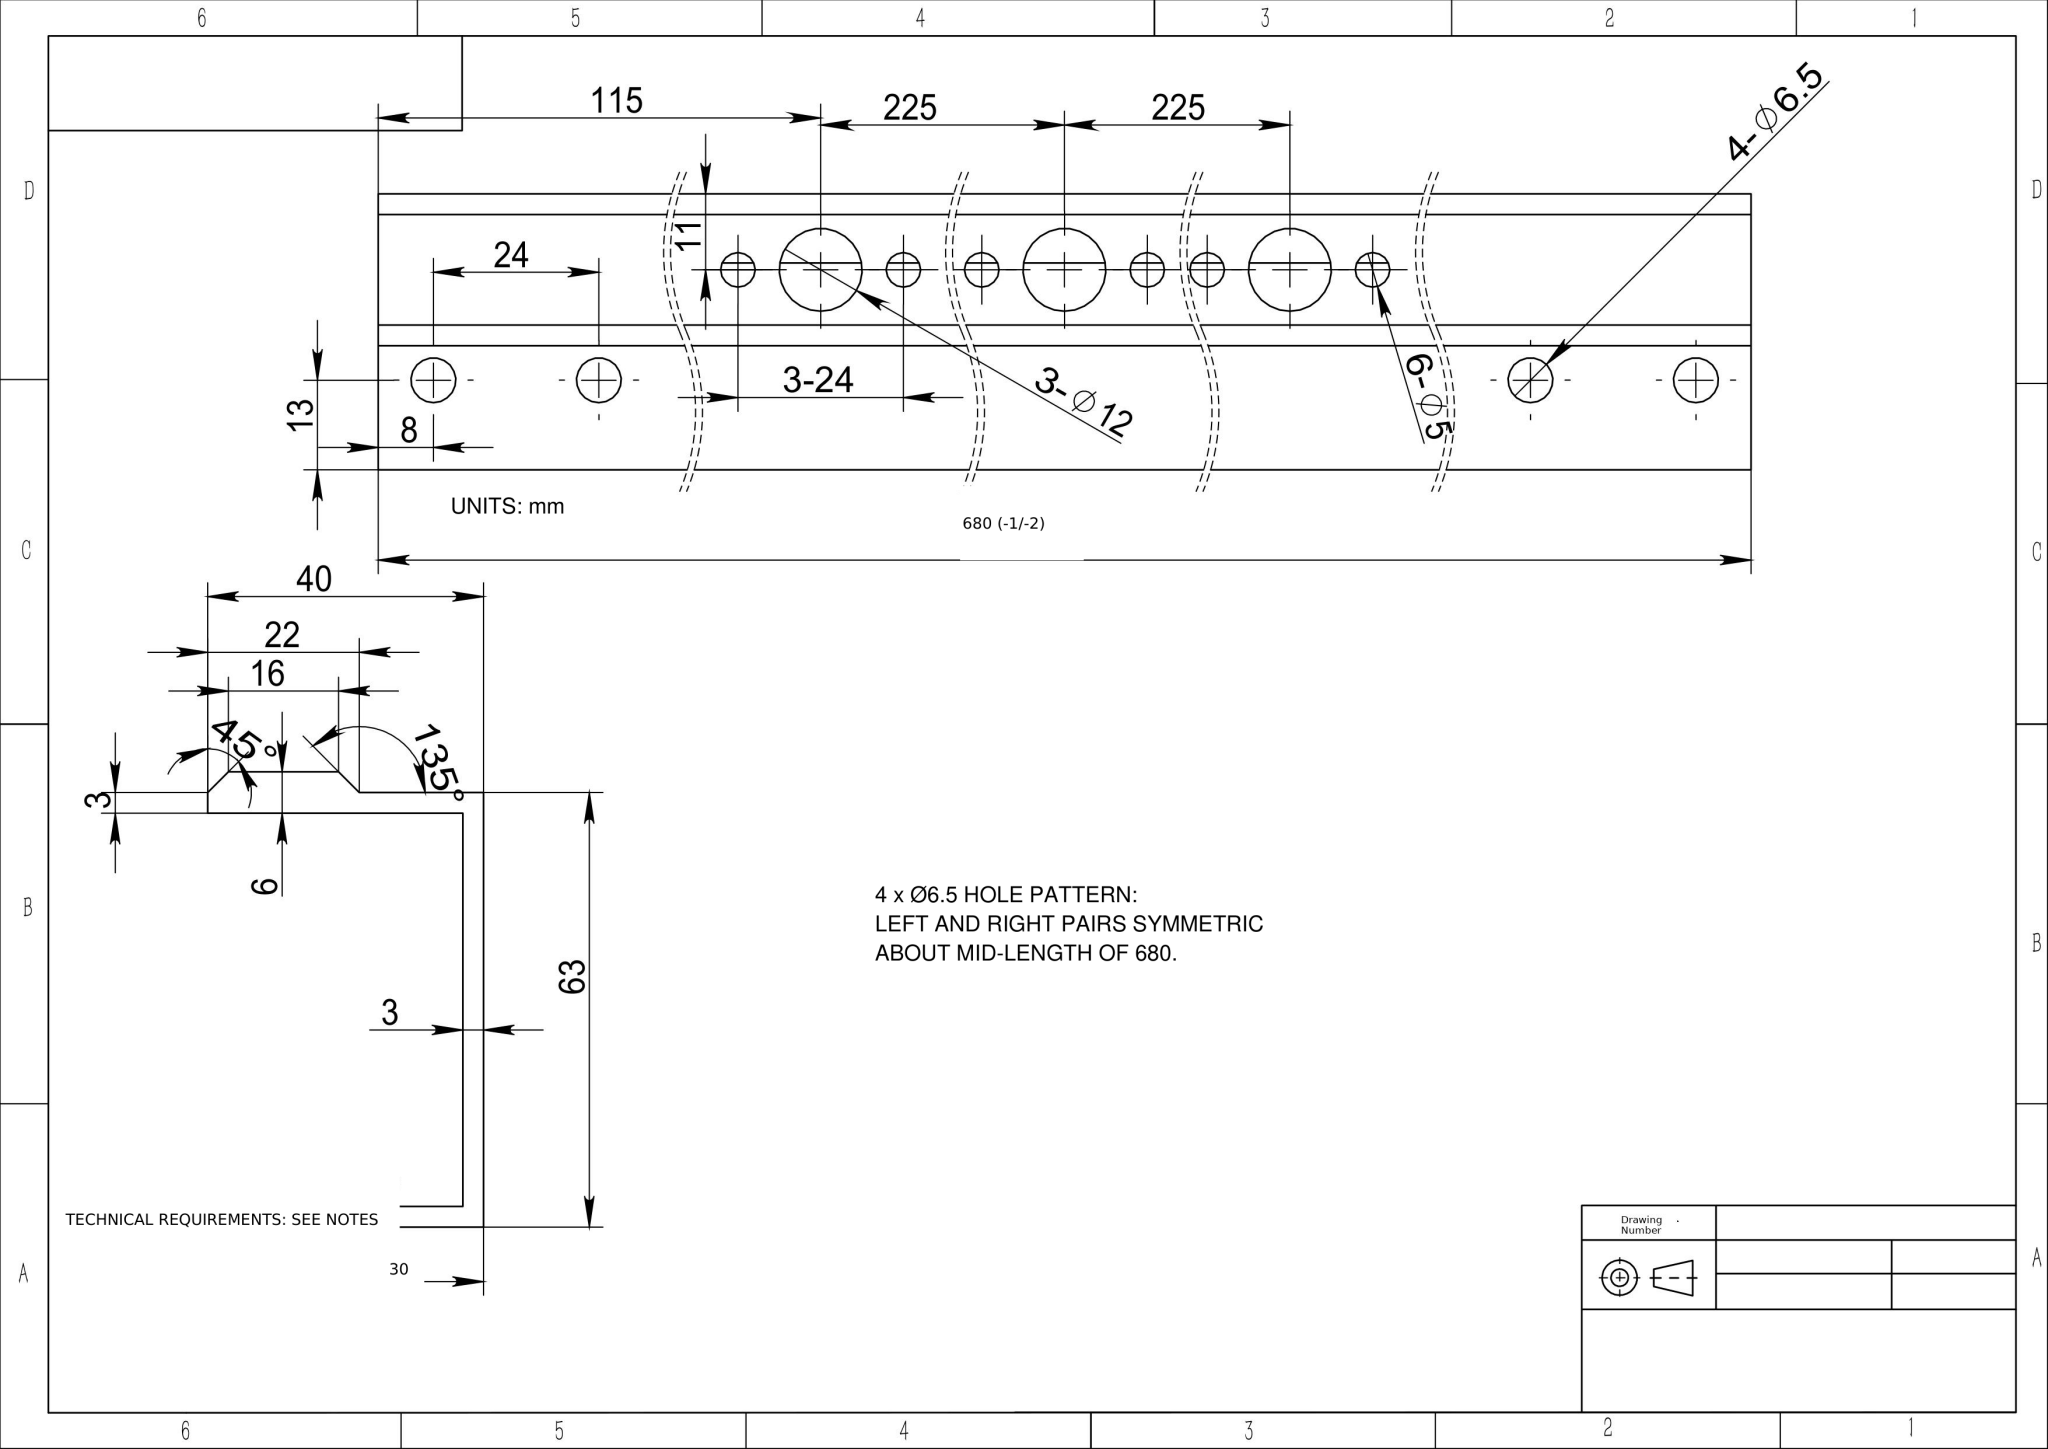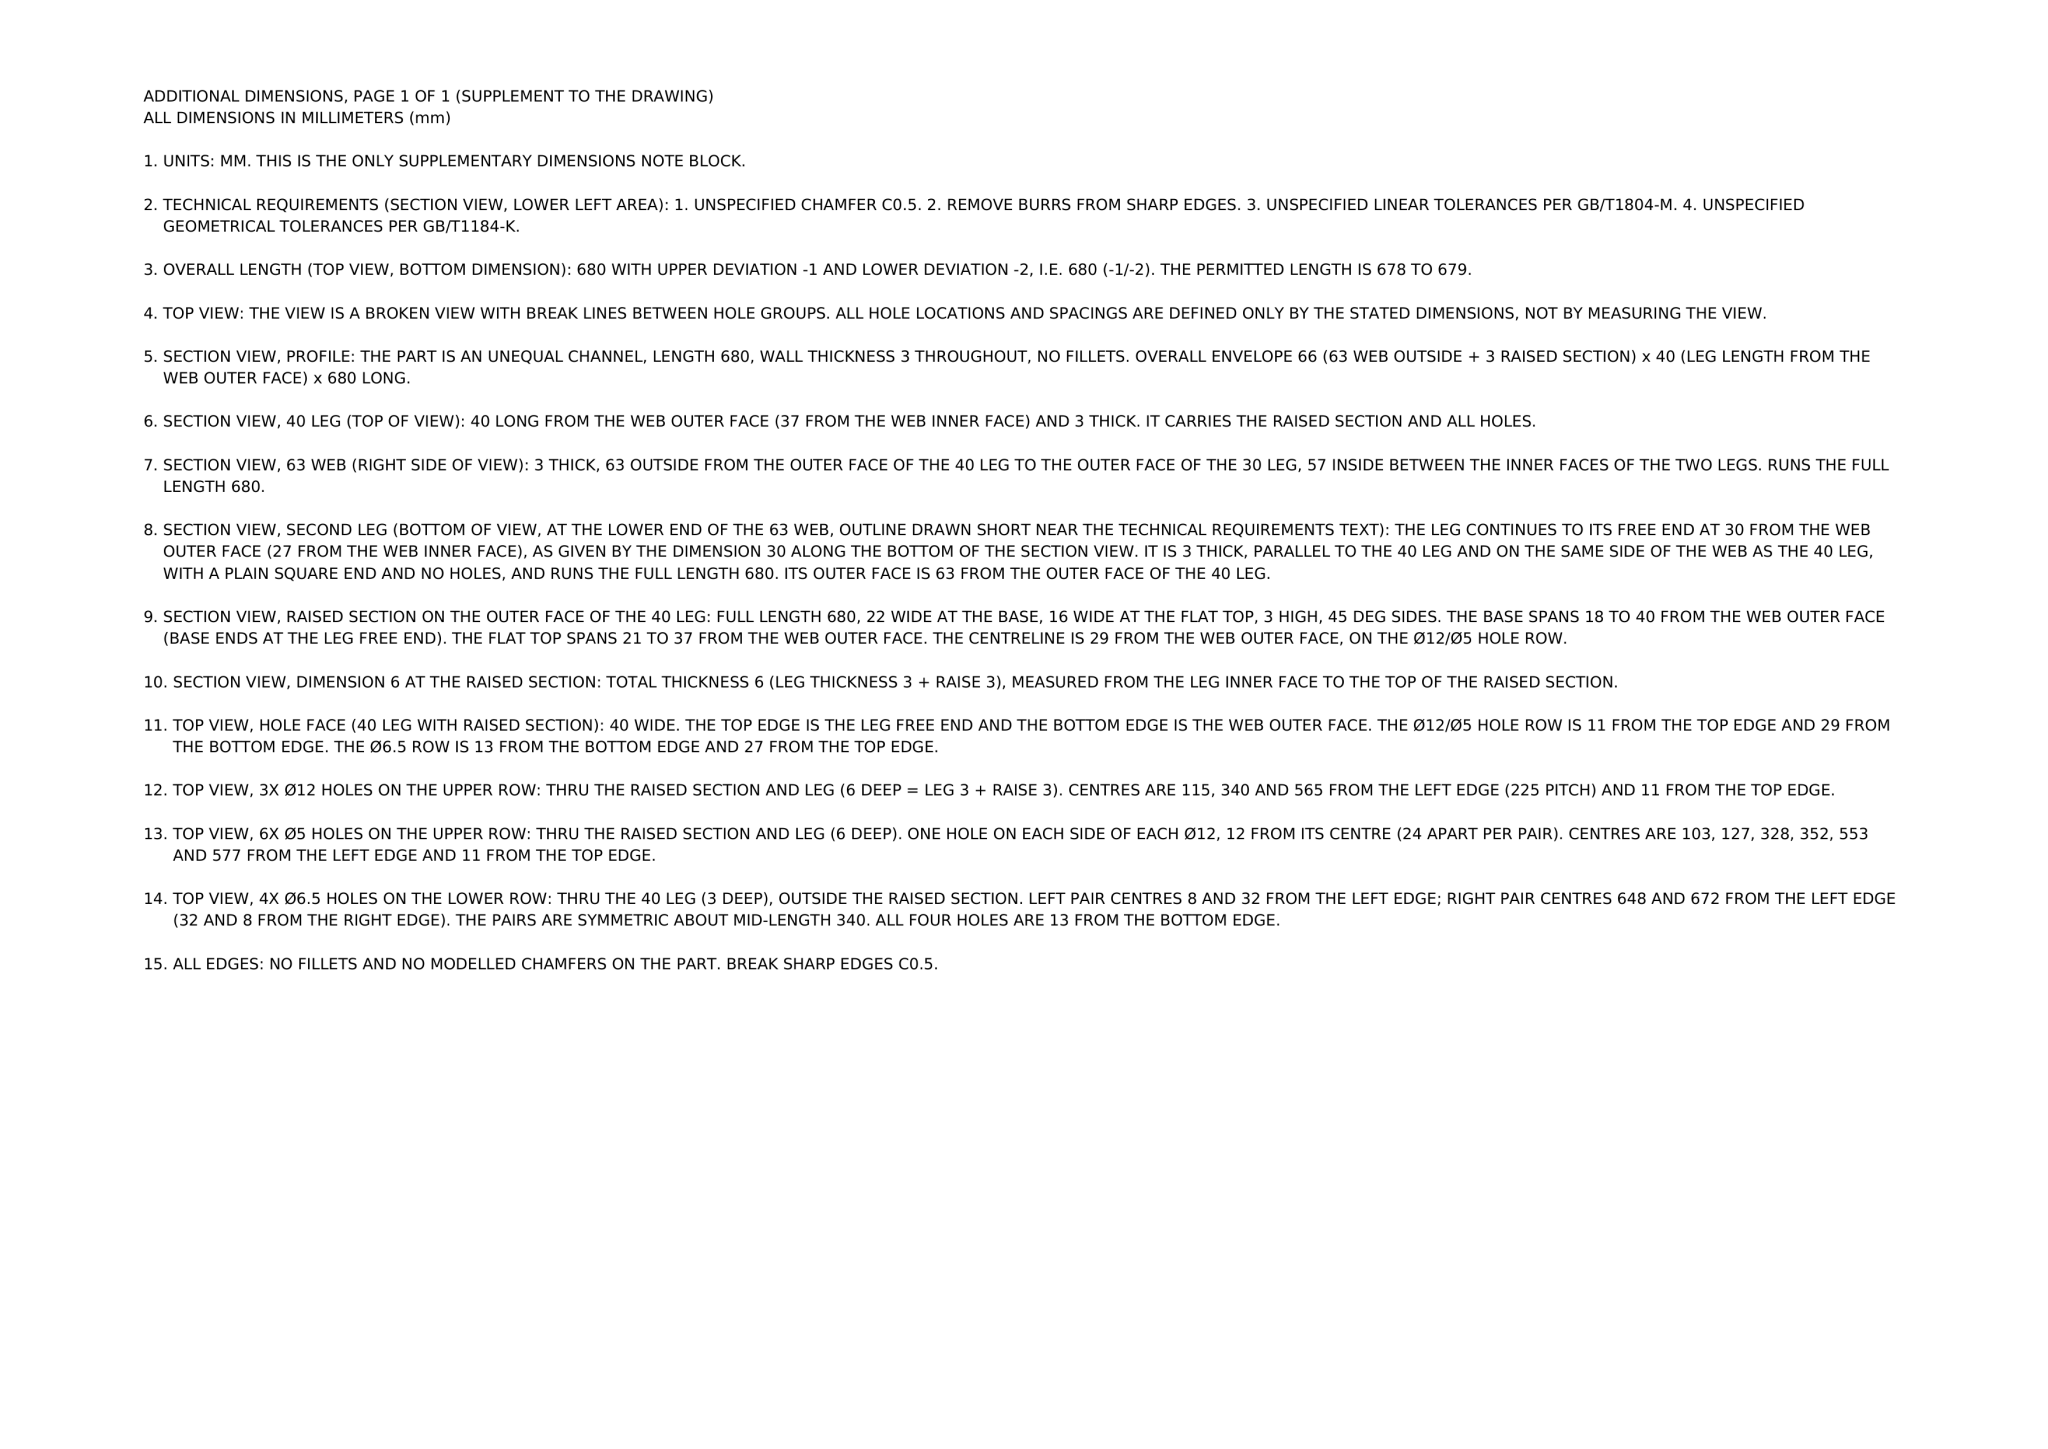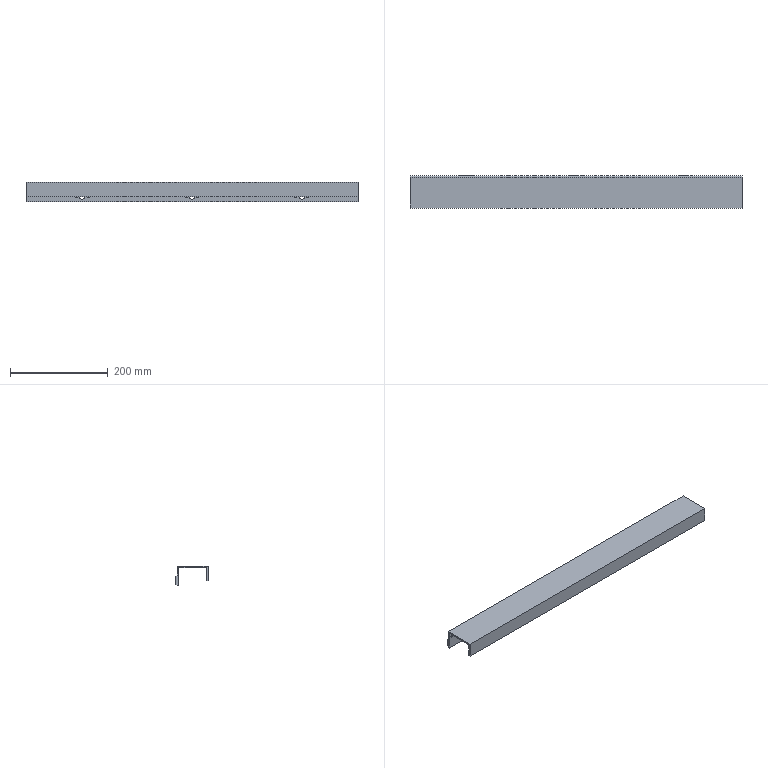Part | NX | mm | 1 solid | 39 faces | box 680 x 66 x 40 mm | volume 294699 mm3 | cylinder 26 | plane 13 | commonest cylinder face diameters 5 x12 6.5 x8 12 x6